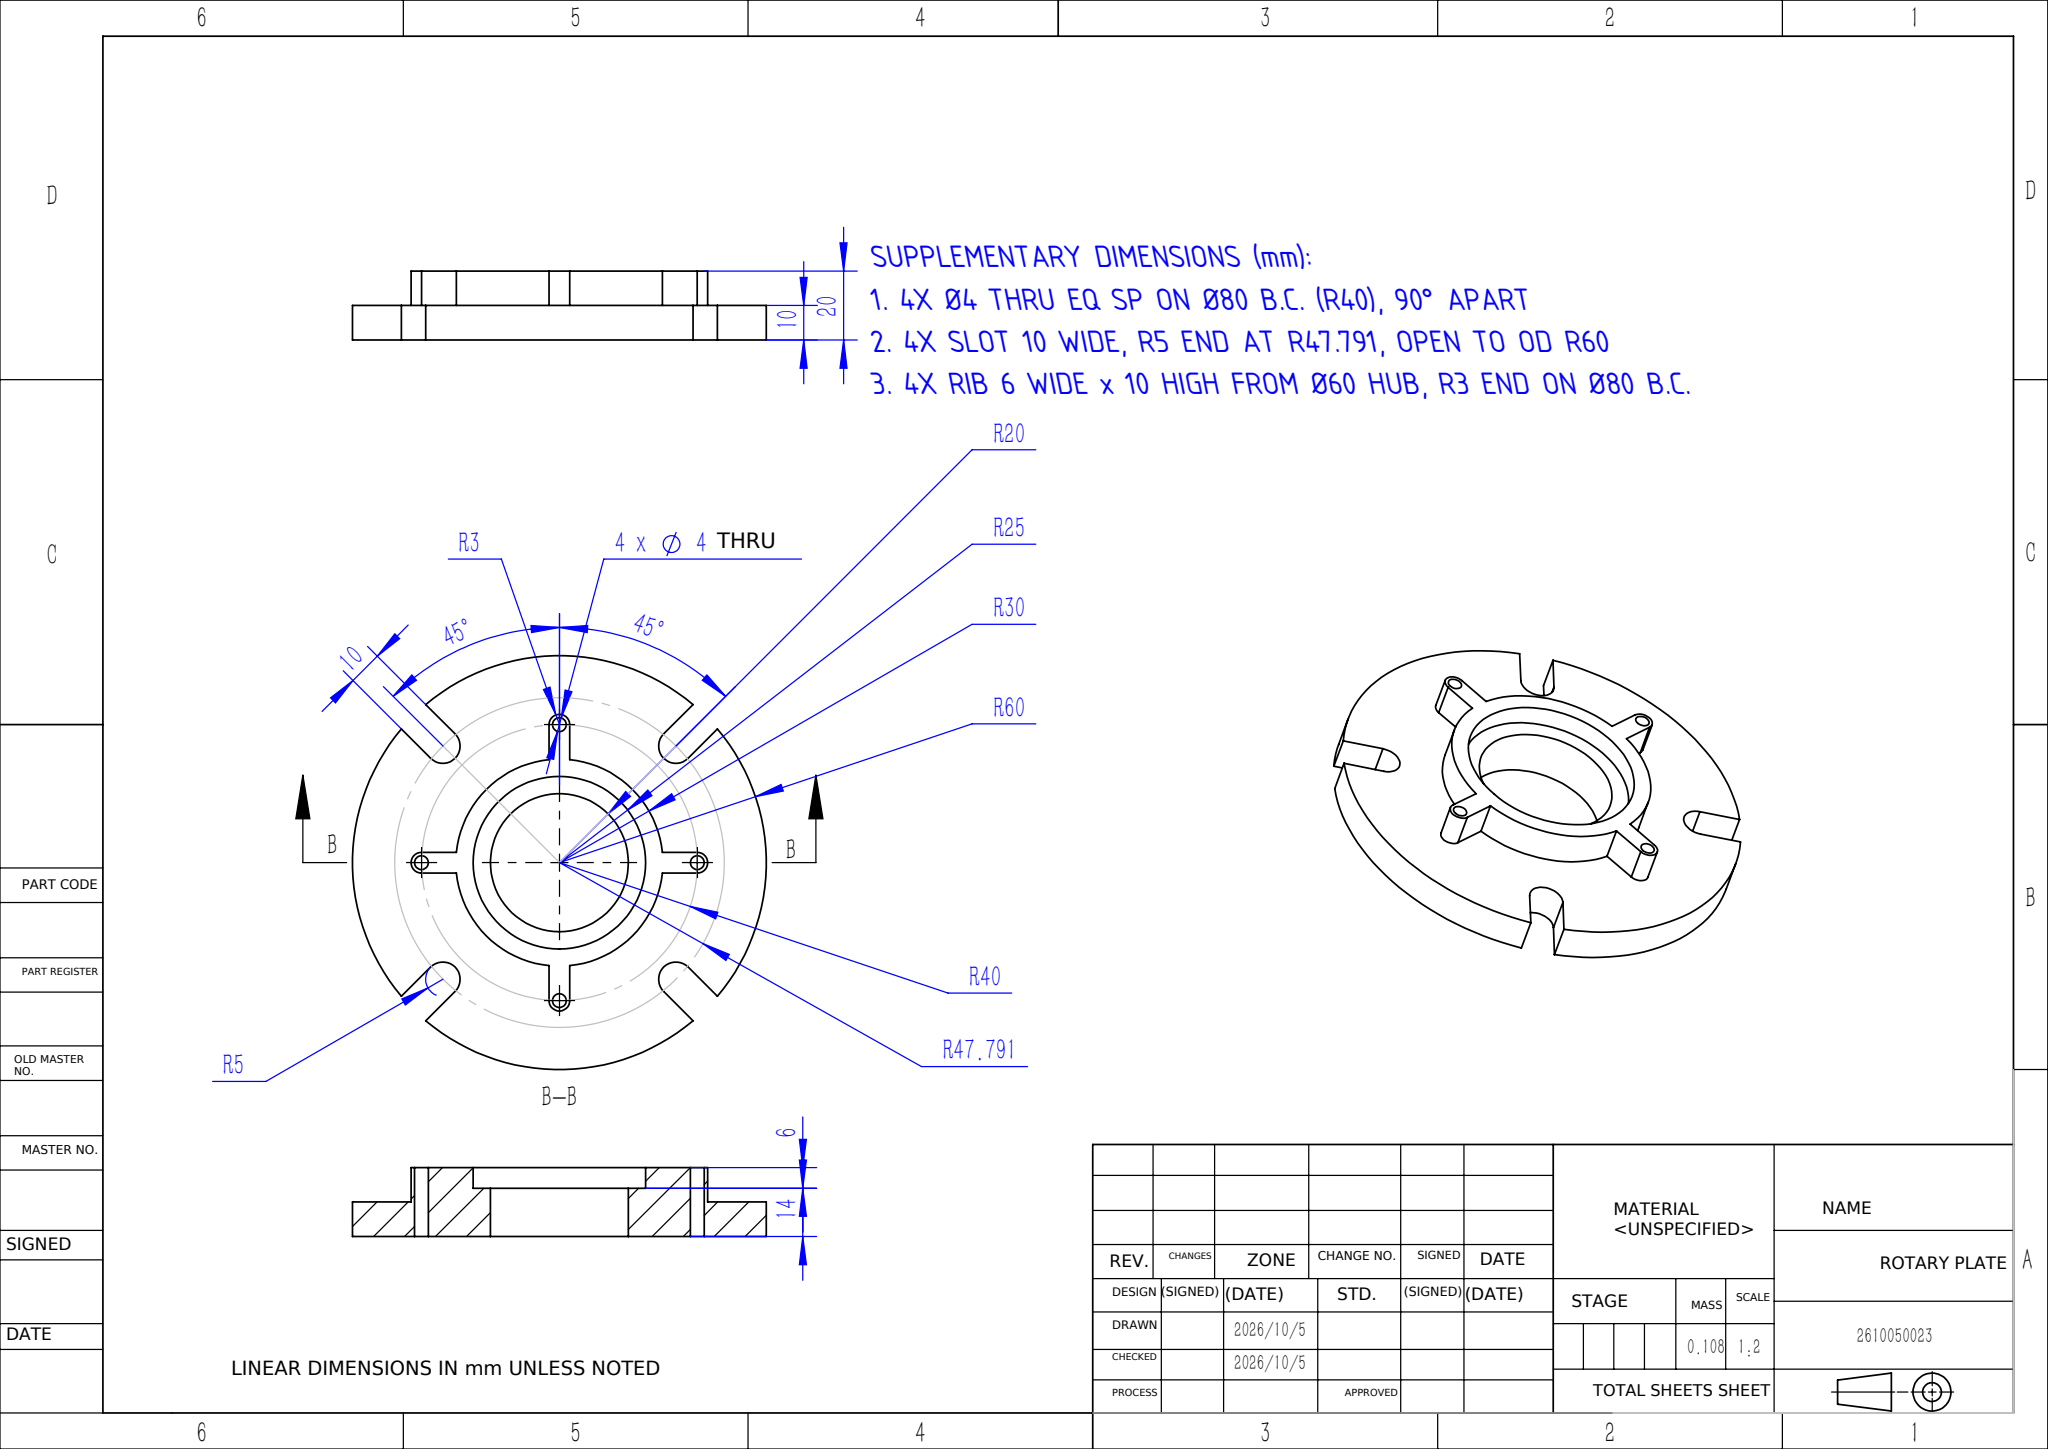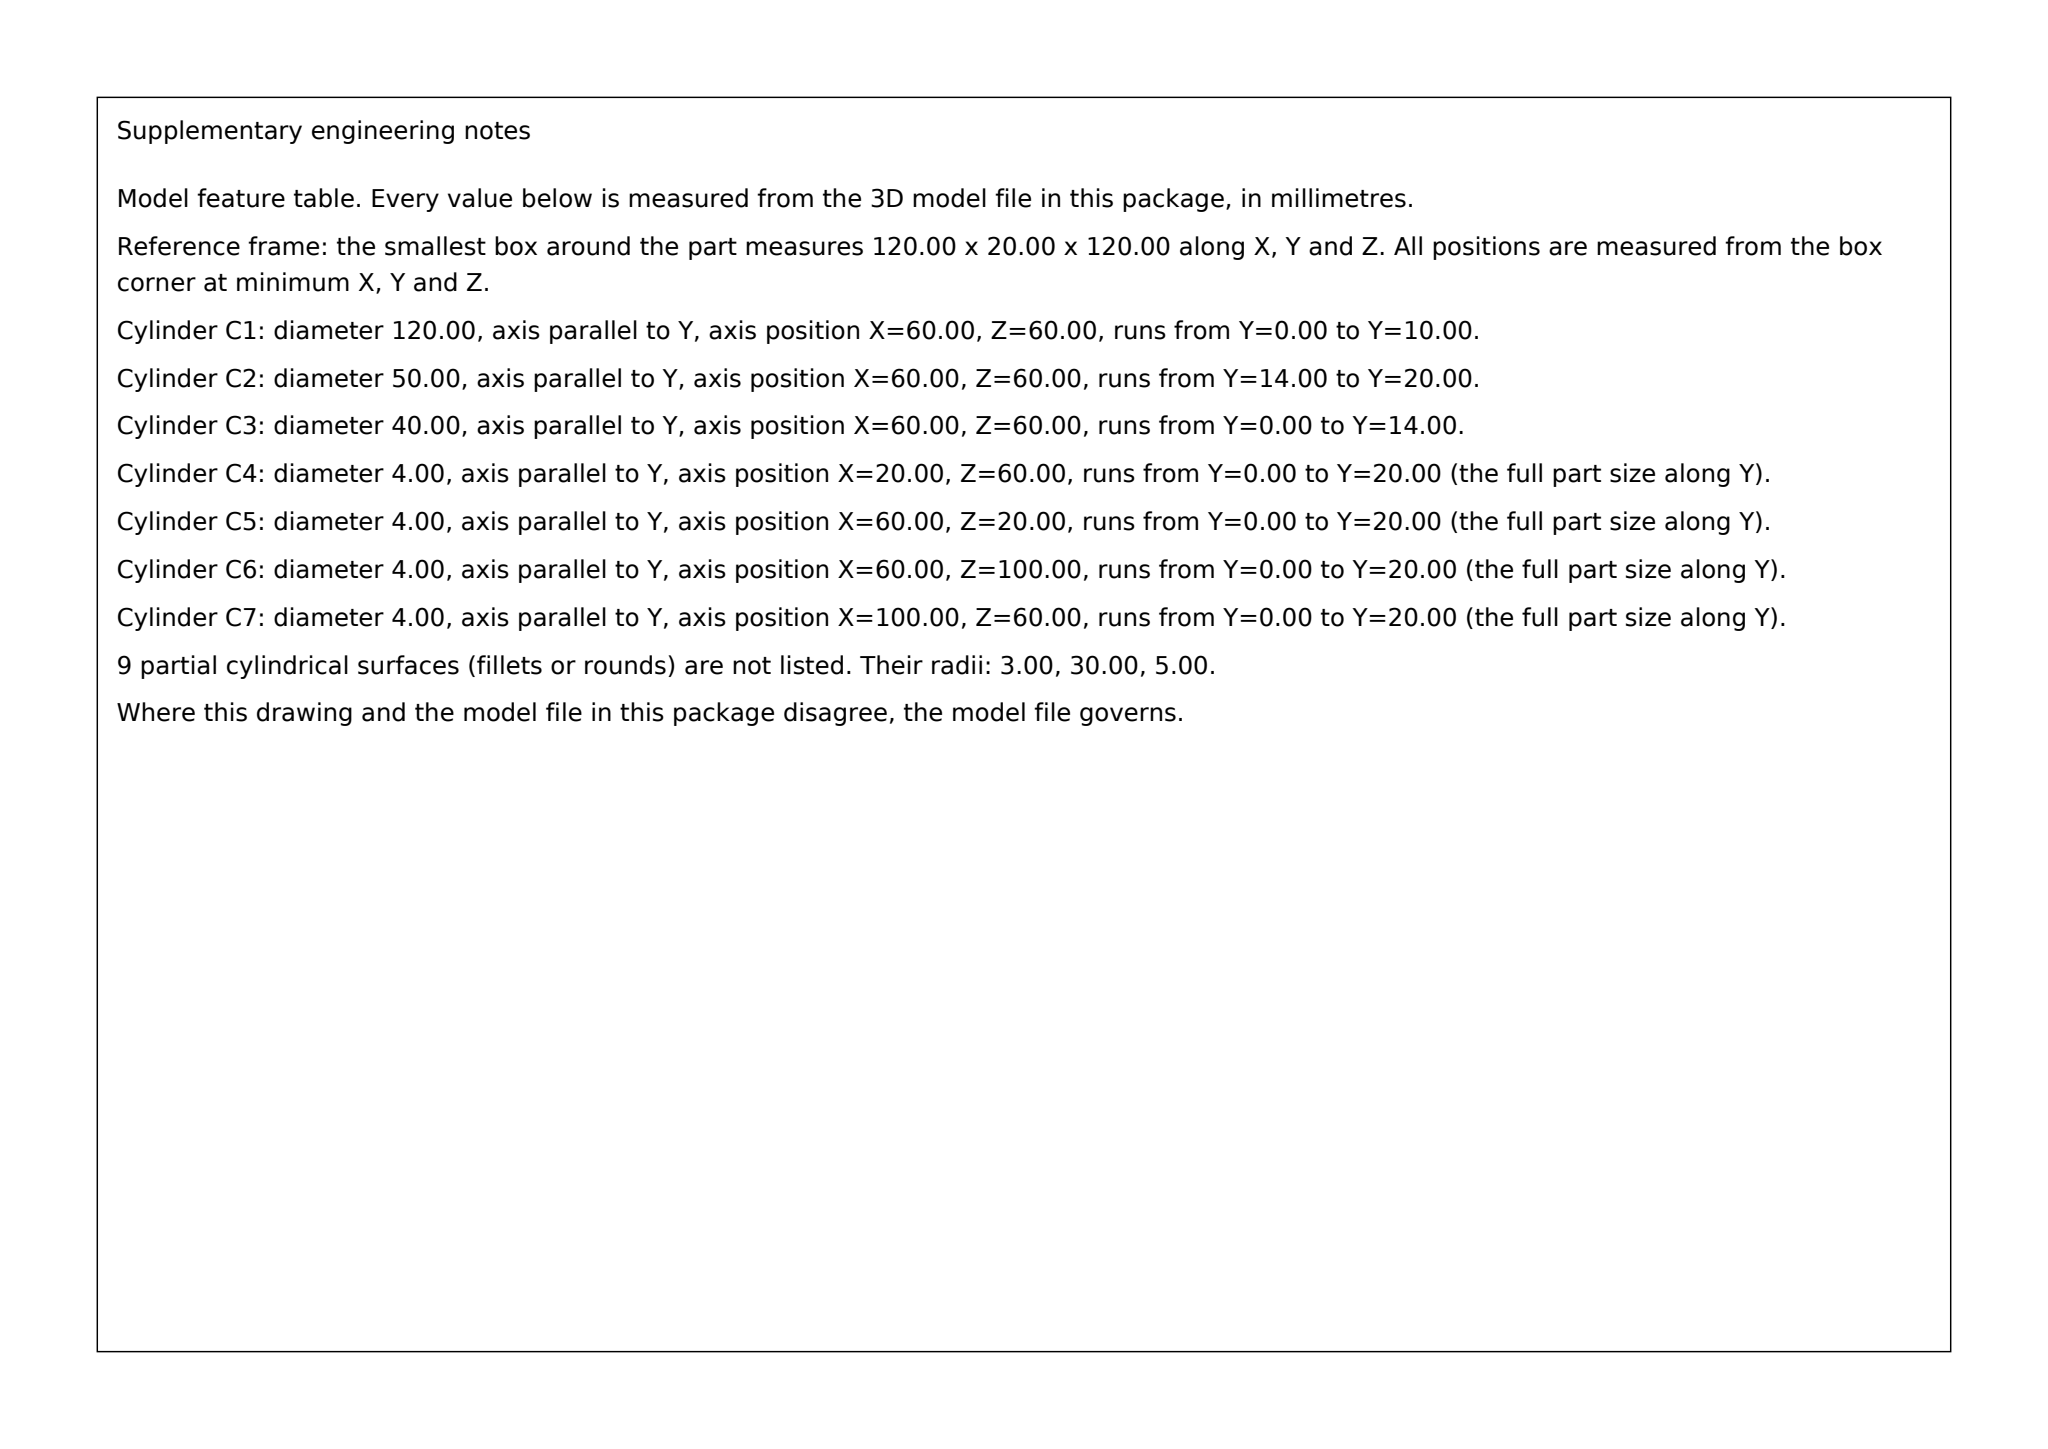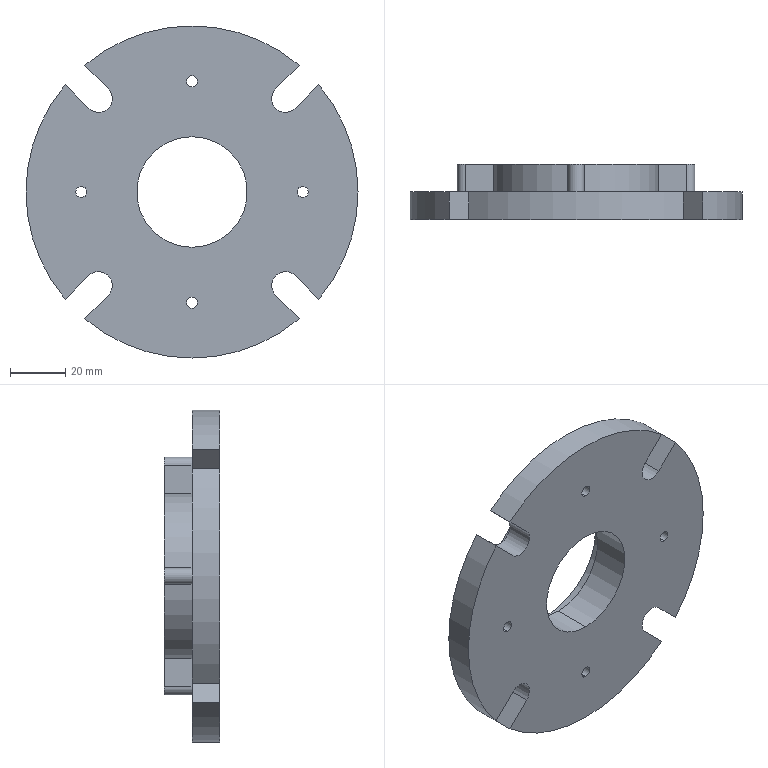Part | SolidWorks | mm | 1 solid | 52 faces | box 120 x 20 x 120 mm | volume 107544 mm3 | cylinder 32 | plane 20 | commonest cylinder face diameters 4 x8 10 x6 6 x5 120 x5 60 x4 50 x2 40 x2